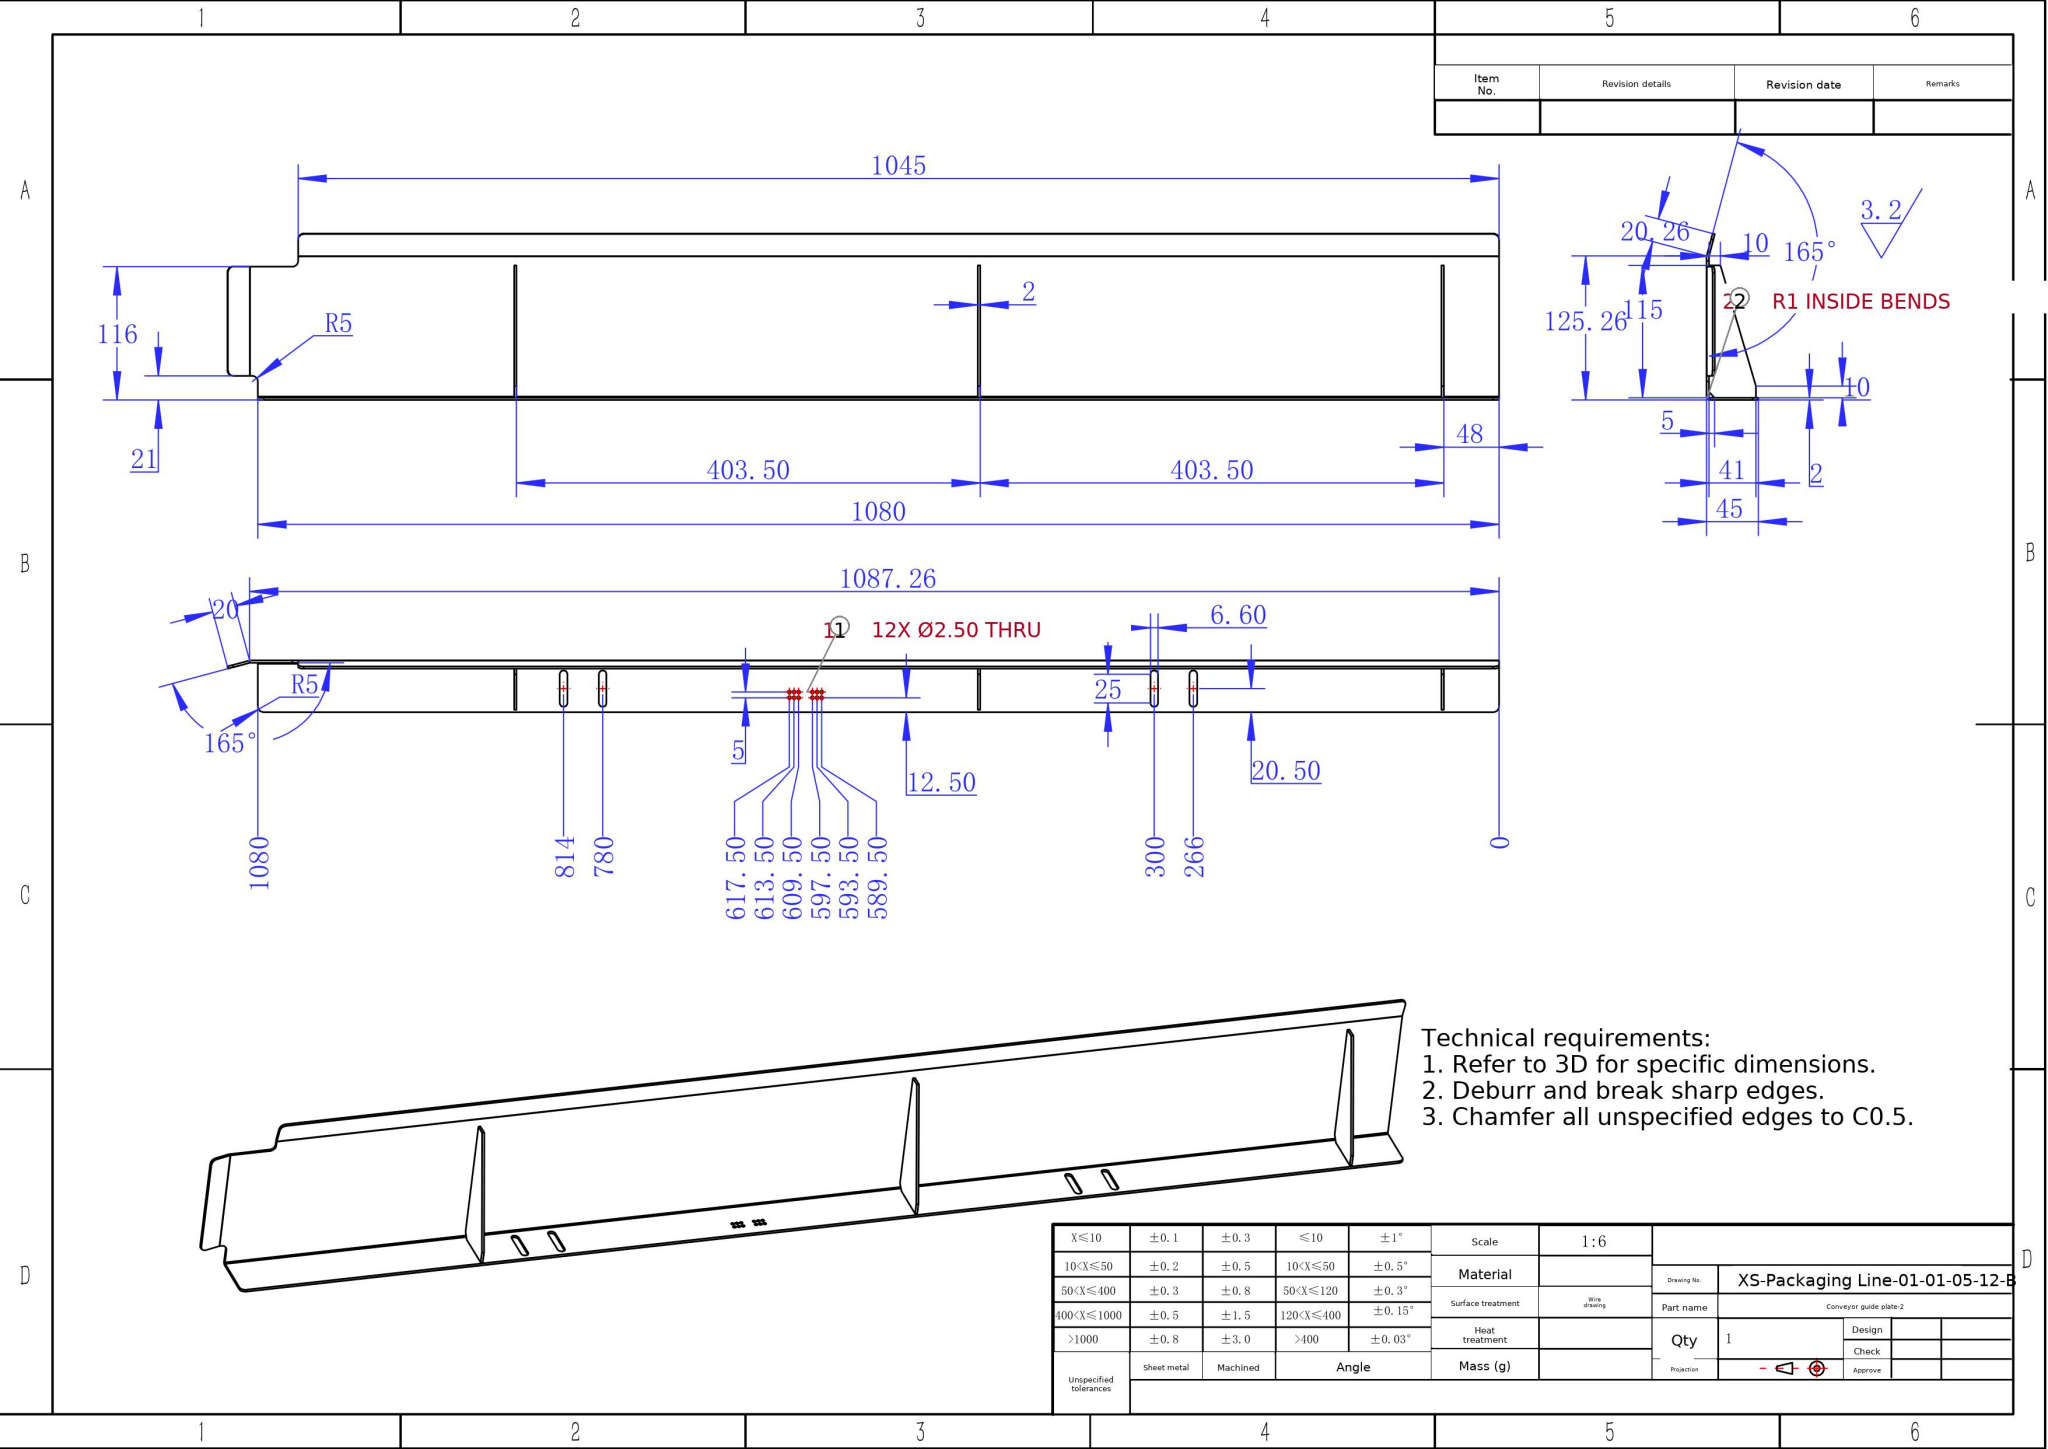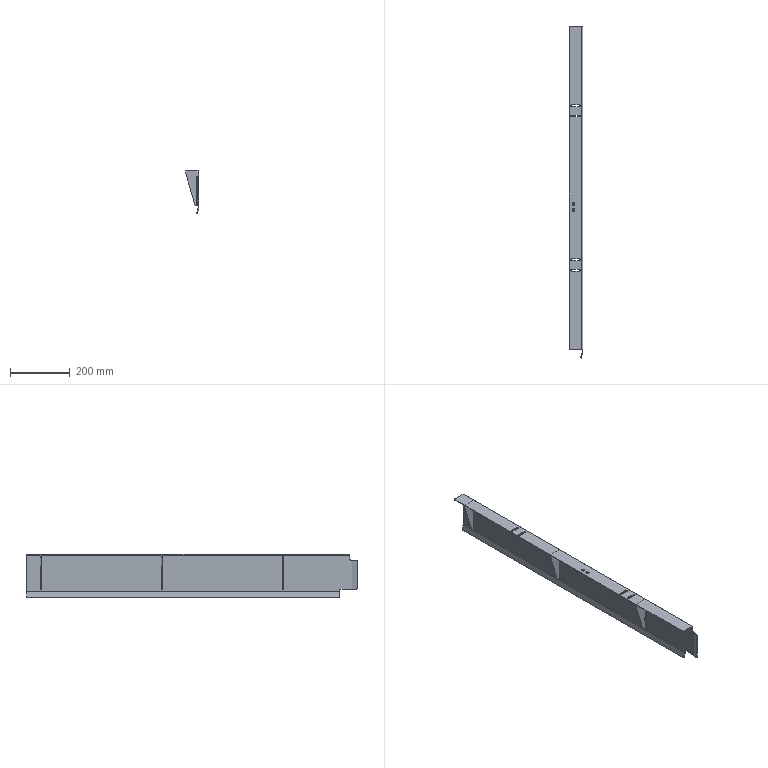Part | SolidWorks | mm | 1 solid | 102 faces | box 45 x 1106.58 x 144.84 mm | volume 424565 mm3 | plane 52 | cylinder 50 | commonest cylinder face diameters 2.5 x24 6.6 x12 10 x8 2 x3 6 x3